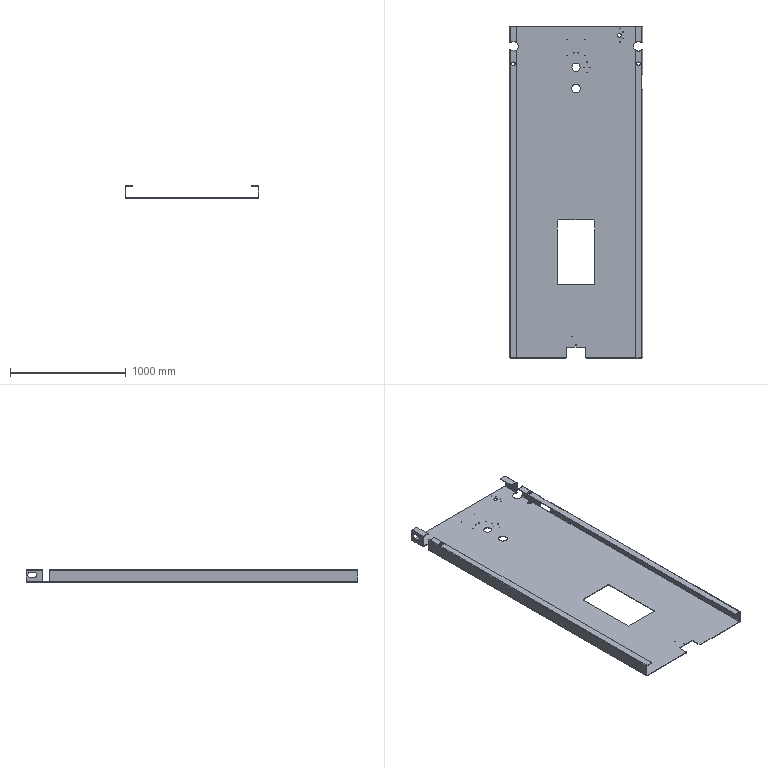Component | SolidWorks | BodyMainBoard-1 | 1 solid | 178 faces | volume 19796460 mm3 | plane 90 | cylinder 83 | spline 5 | commonest cylinder face diameters 5.2 x16 8 x13 18 x9 5 x8 32.5 x4 30 x4 6.8 x4 20 x4 | material Q235